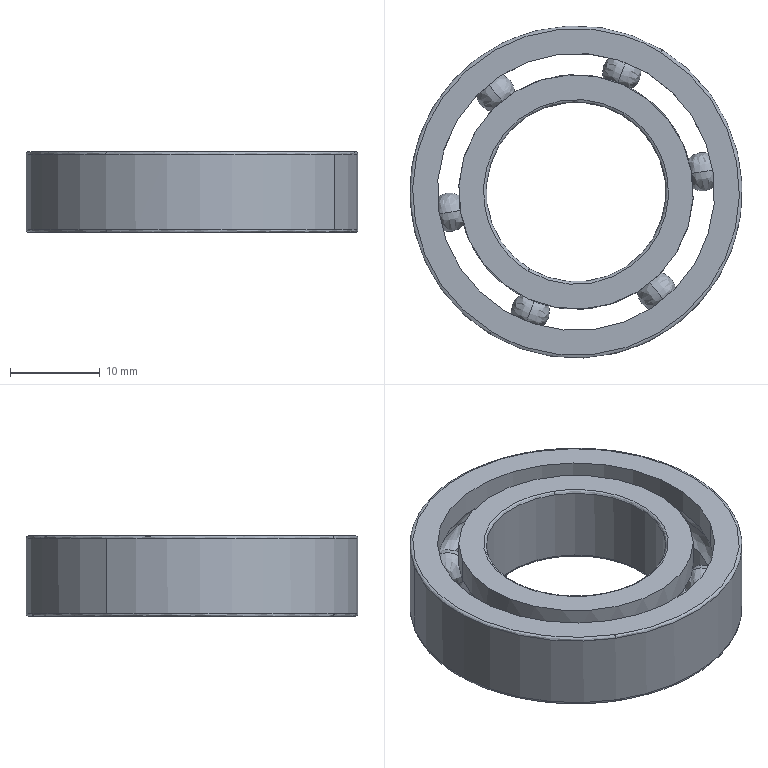Component | SolidWorks | 61904Bearing-2 | 8 solids | 42 faces | volume 4751 mm3 | spline 26 | cylinder 12 | plane 4 | commonest cylinder face diameters 26.12 x4 30.88 x4 20 x2 37 x2 | material 45#Steel